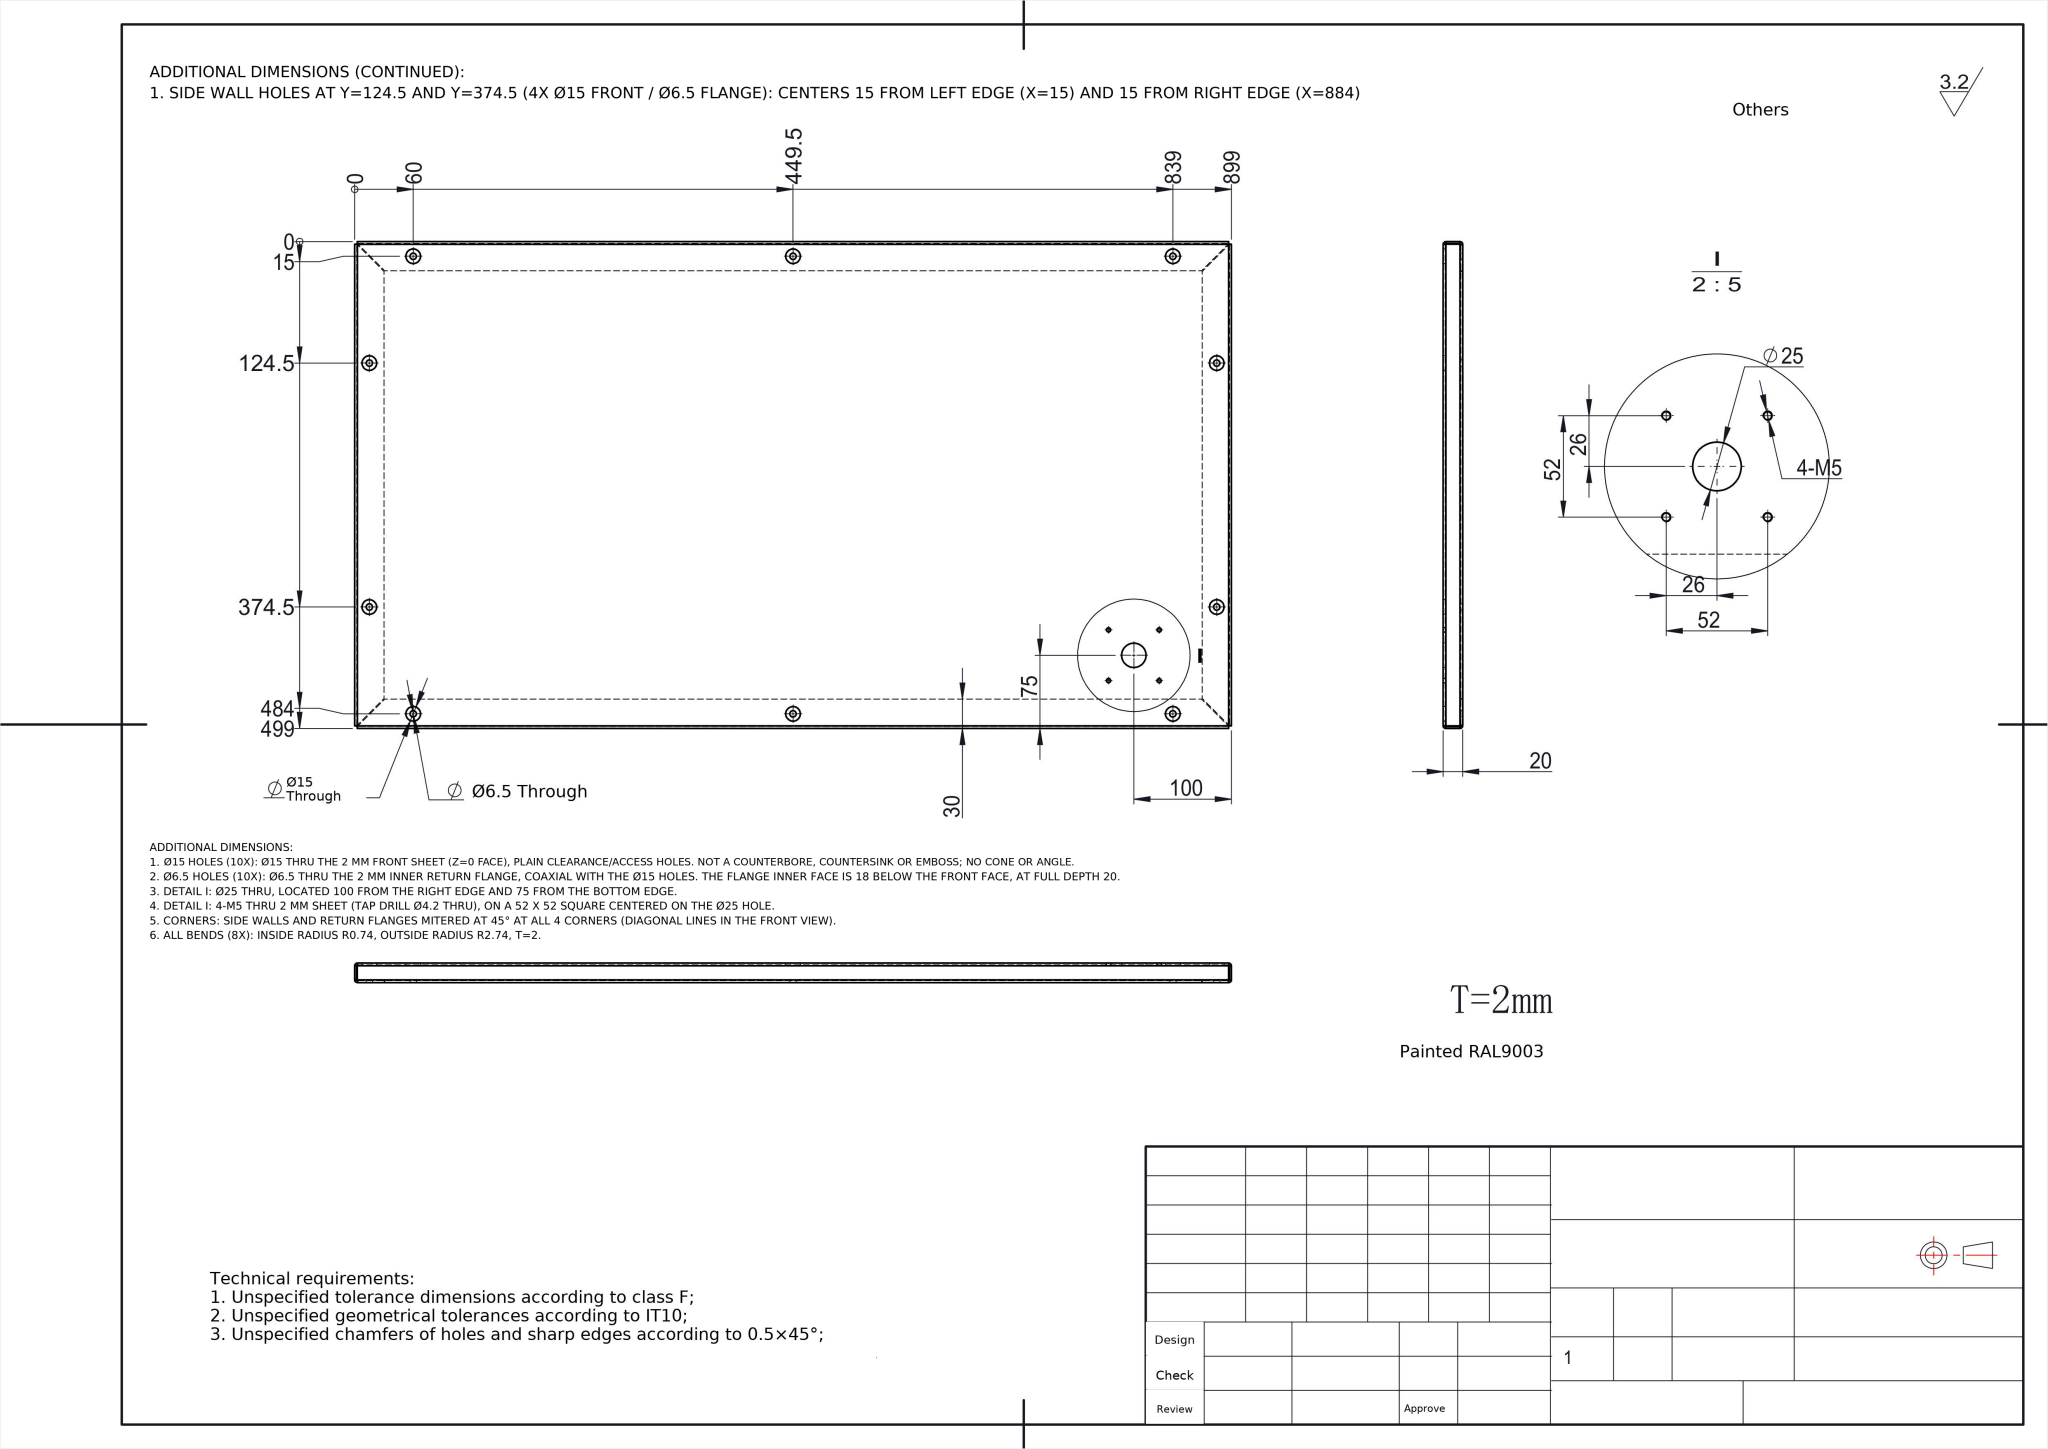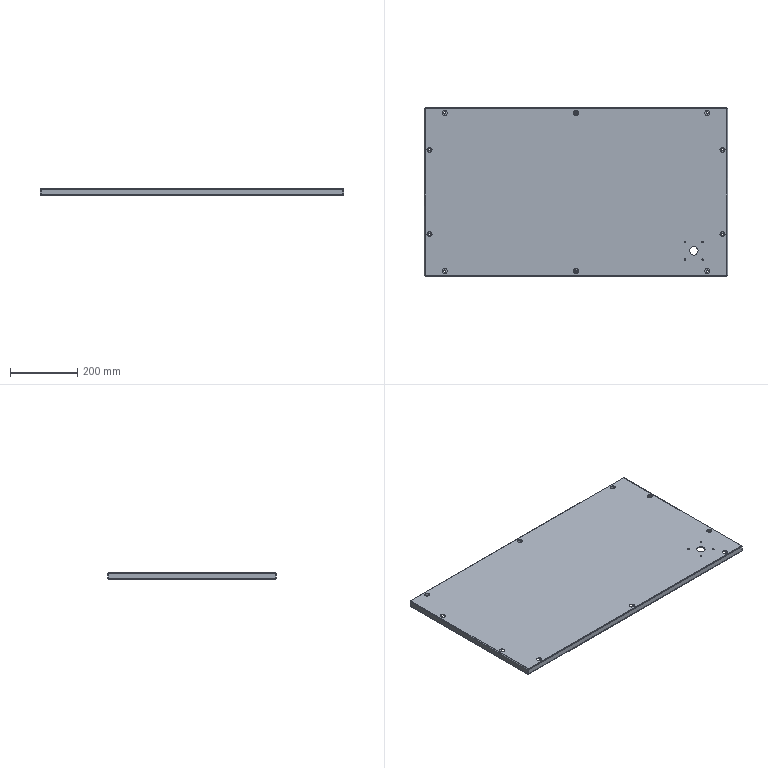Part | NX | mm | 1 solid | 120 faces | box 899 x 499 x 20 mm | volume 1132537 mm3 | cylinder 66 | plane 38 | spline 16 | commonest cylinder face diameters 15 x20 6.5 x20 4.2 x8 5.473 x8 1.473 x8 25 x2